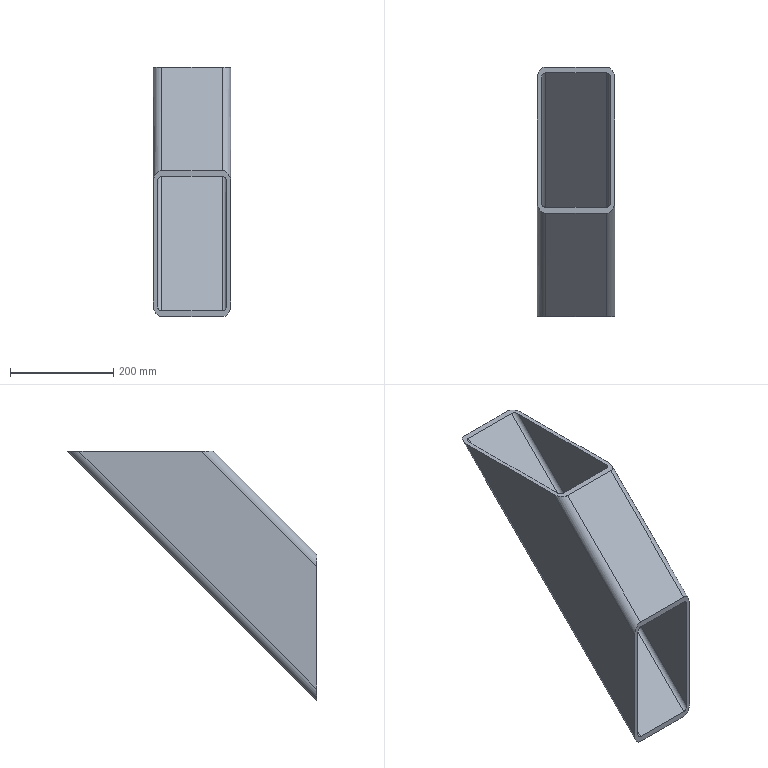Component | NX | AAAAAAAAAAAAAAAAAAAAAAAAAAAAAAAAAAAAAAAAAAAAAAAAAAAAAAAAAAA_3 | 1 solid | 18 faces | volume 2500732 mm3 | plane 10 | cylinder 8 | commonest cylinder face diameters 32 x4 16 x4